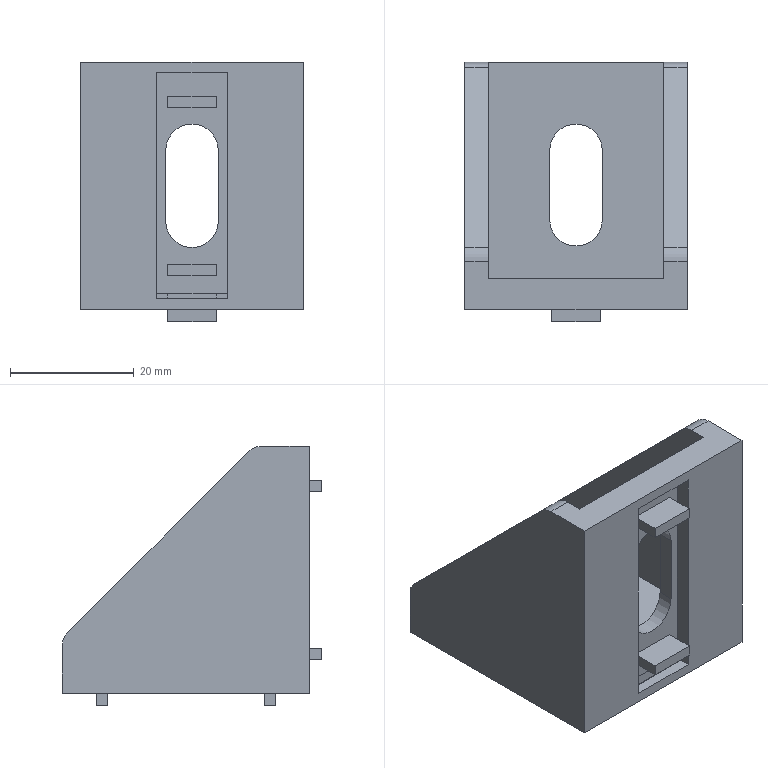Component | SolidWorks | ABB11-G408-4040AngleBracket-55 | 1 solid | 52 faces | volume 16562 mm3 | plane 44 | cylinder 8 | commonest cylinder face diameters 8.5 x4 6 x4